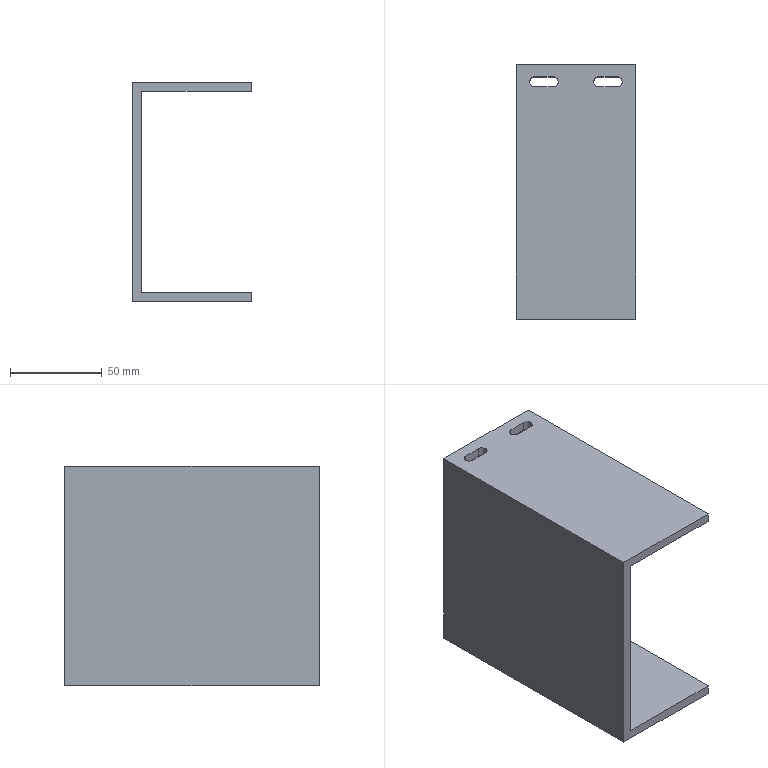Component | SolidWorks | F9-1 | 1 solid | 30 faces | box 65 x 139 x 120 mm | volume 165225 mm3 | plane 18 | cylinder 12 | commonest cylinder face diameters 5.5 x12
build123d program:
from build123d import *

# Parameters (mm, degrees)
EXTRUDE_THIN1_DEPTH = 139
CUT_EXTRUDE1_DEPTH  = 248.168


with BuildPart() as part:
    # Sketch1 → Extrude-Thin1 (new body)
    with BuildSketch(Plane.XY):
        Polygon((0, 100.441), (0, 160.441), (110, 160.441), (110, 100.441), (115, 100.441), (115, 165.441), (-5, 165.441), (-5, 100.441), align=None)
    extrude(amount=EXTRUDE_THIN1_DEPTH)

    # Sketch2 → Cut-Extrude1 (cut, through all)
    with BuildSketch(Plane(origin=(115, 0, 0), x_dir=(0, 0, -1), z_dir=(1, 0, 0))):
        with BuildLine():
            Line((-126.796, 155.441), (-126.796, 145.441))
            ThreePointArc((-126.796, 145.441), (-129.546, 142.691), (-132.296, 145.441))
            Line((-132.296, 145.441), (-132.296, 155.441))
            ThreePointArc((-132.296, 155.441), (-129.546, 158.191), (-126.796, 155.441))
        make_face()
        with BuildLine():
            Line((-126.796, 120.441), (-126.796, 110.441))
            ThreePointArc((-126.796, 110.441), (-129.546, 107.691), (-132.296, 110.441))
            Line((-132.296, 110.441), (-132.296, 120.441))
            ThreePointArc((-132.296, 120.441), (-129.546, 123.191), (-126.796, 120.441))
        make_face()
    extrude(amount=-CUT_EXTRUDE1_DEPTH, mode=Mode.SUBTRACT)


solid = part.part

# Placed as in the assembly
solid = solid.moved(Location((-3.959, 178.279, 18), (-90, 0, 90)))